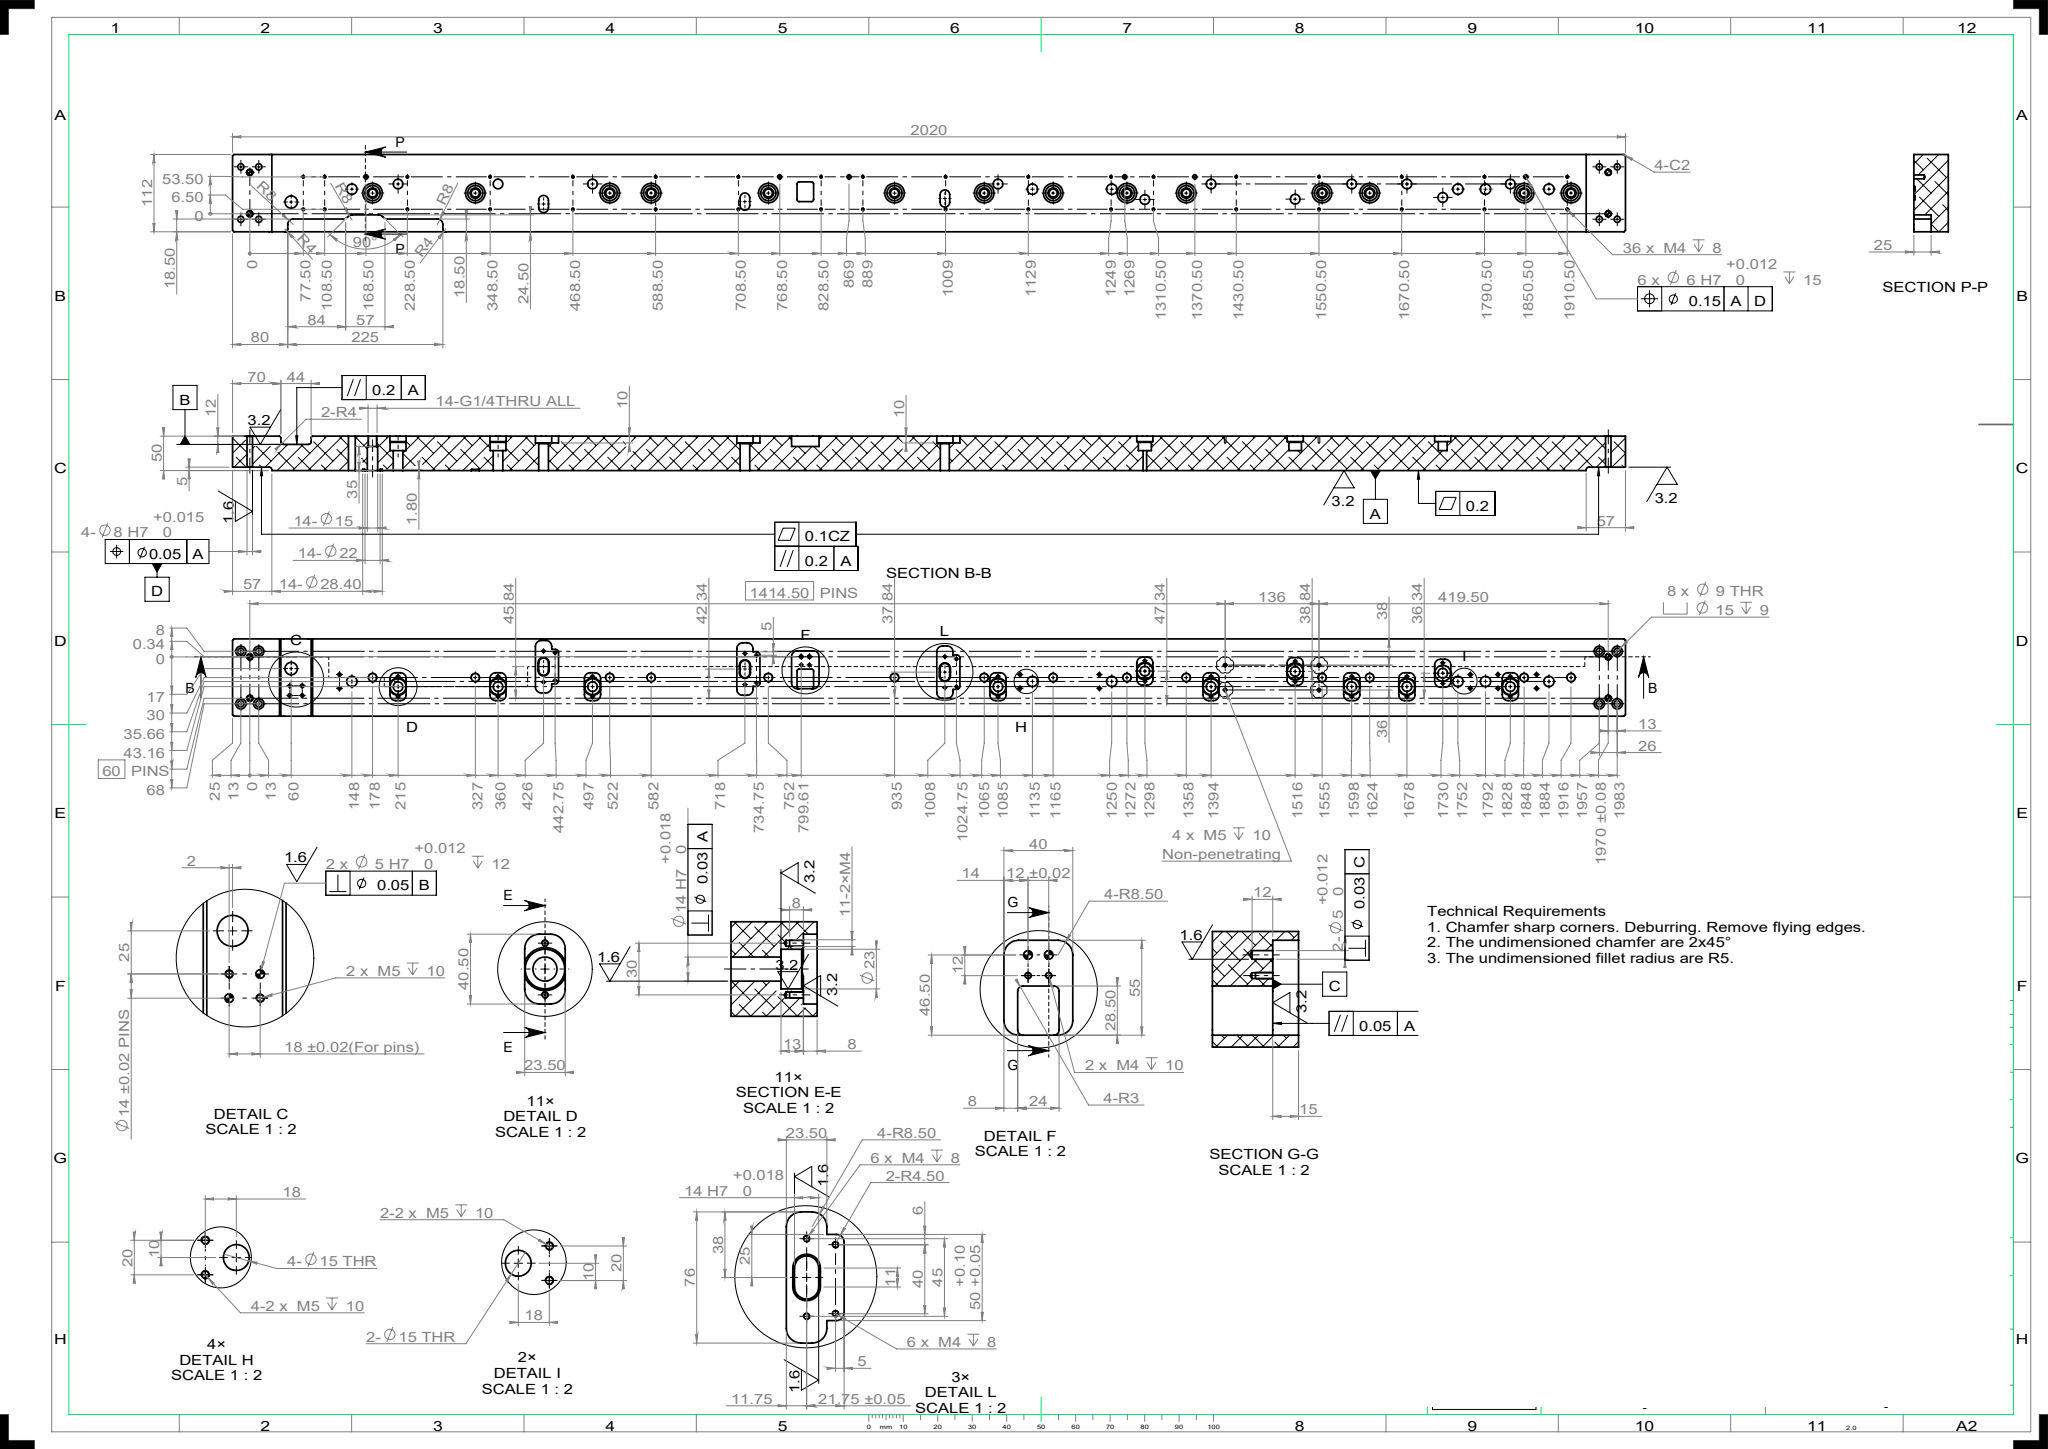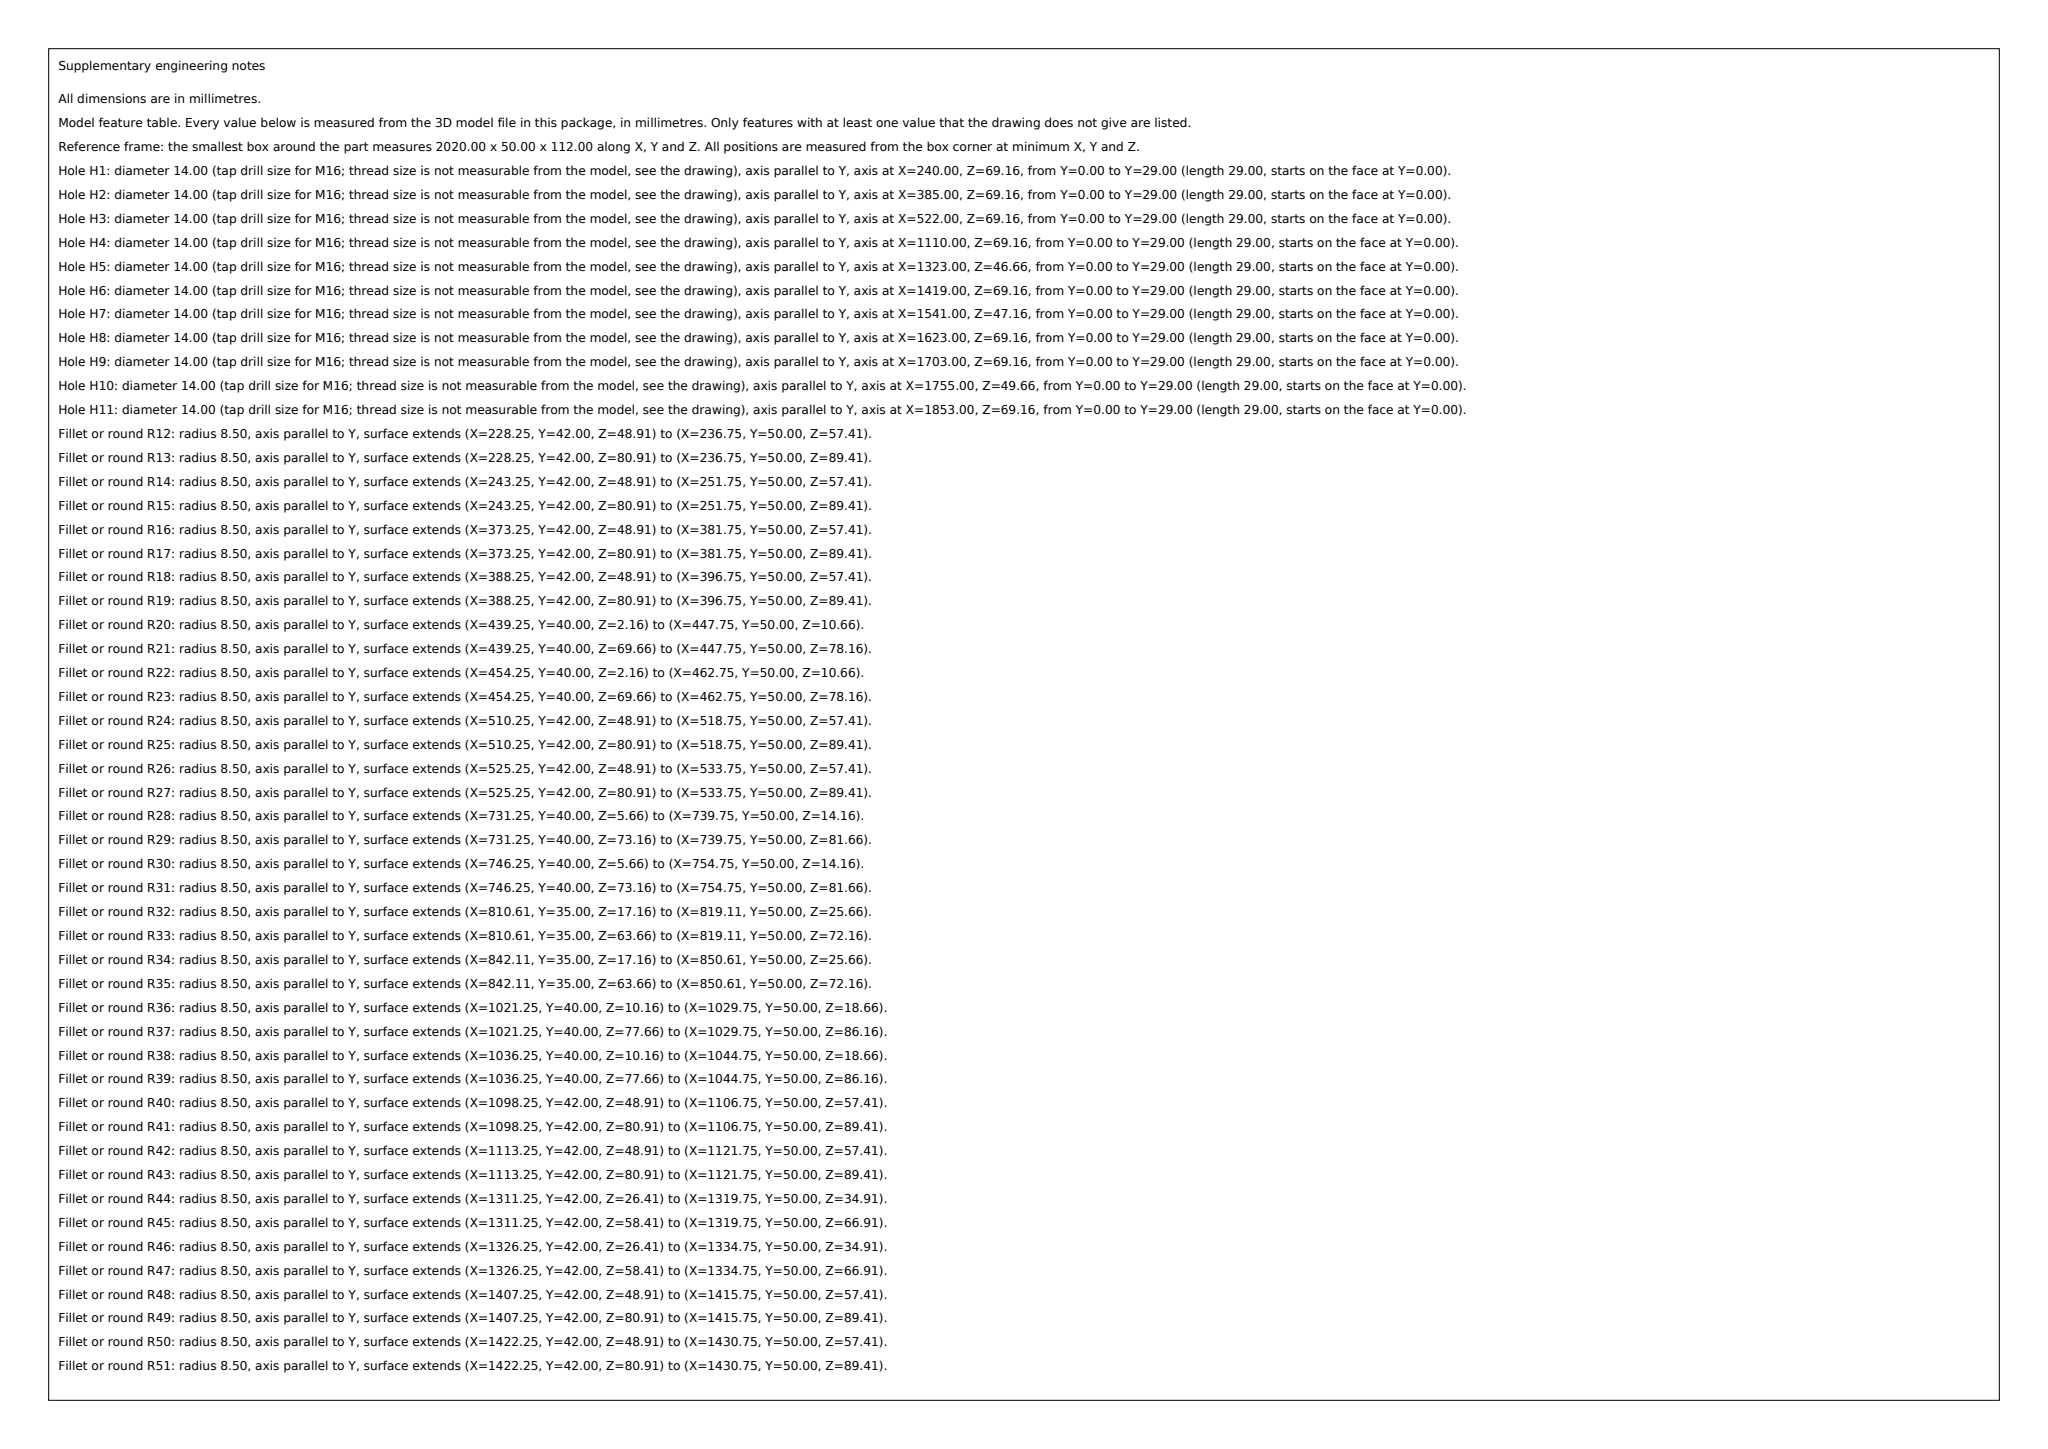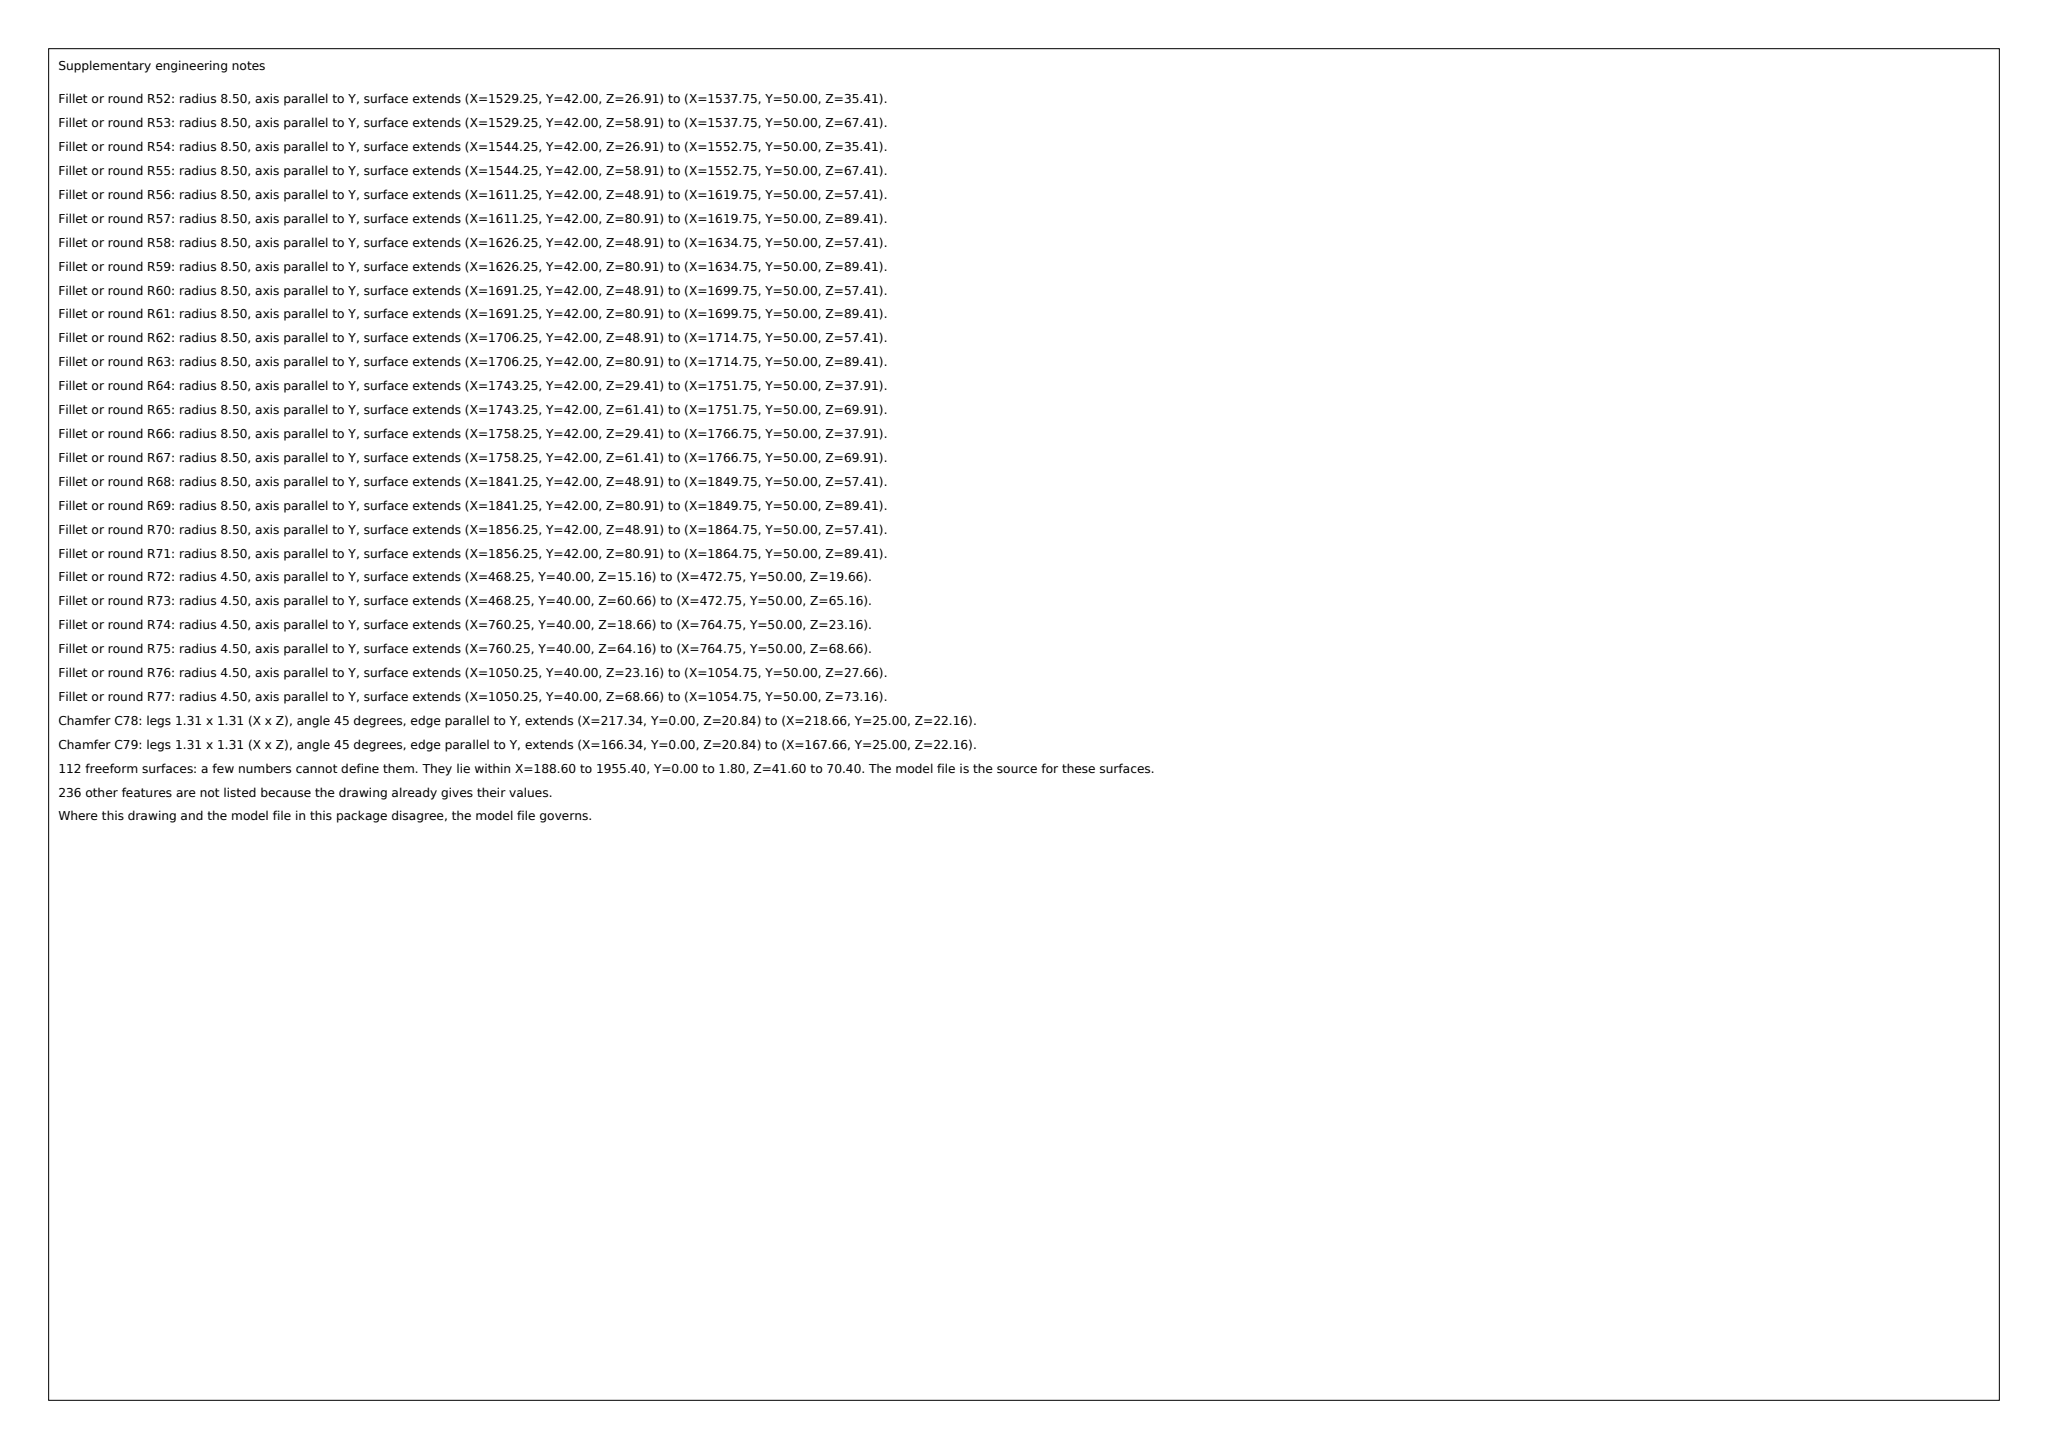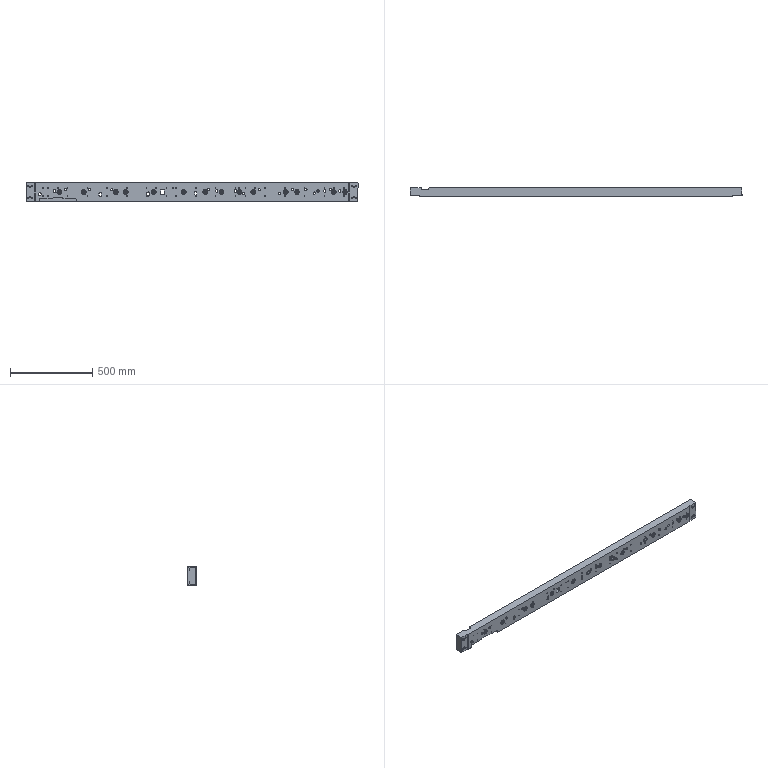Part | SolidWorks | mm | 1 solid | 1050 faces | box 2020 x 50 x 112 mm | volume 10500324 mm3 | cylinder 501 | cone 230 | plane 207 | spline 112 | commonest cylinder face diameters 3.3 x144 17 x60 15 x56 4.2 x36 14 x31 28.4 x28 11.8 x28 22 x28